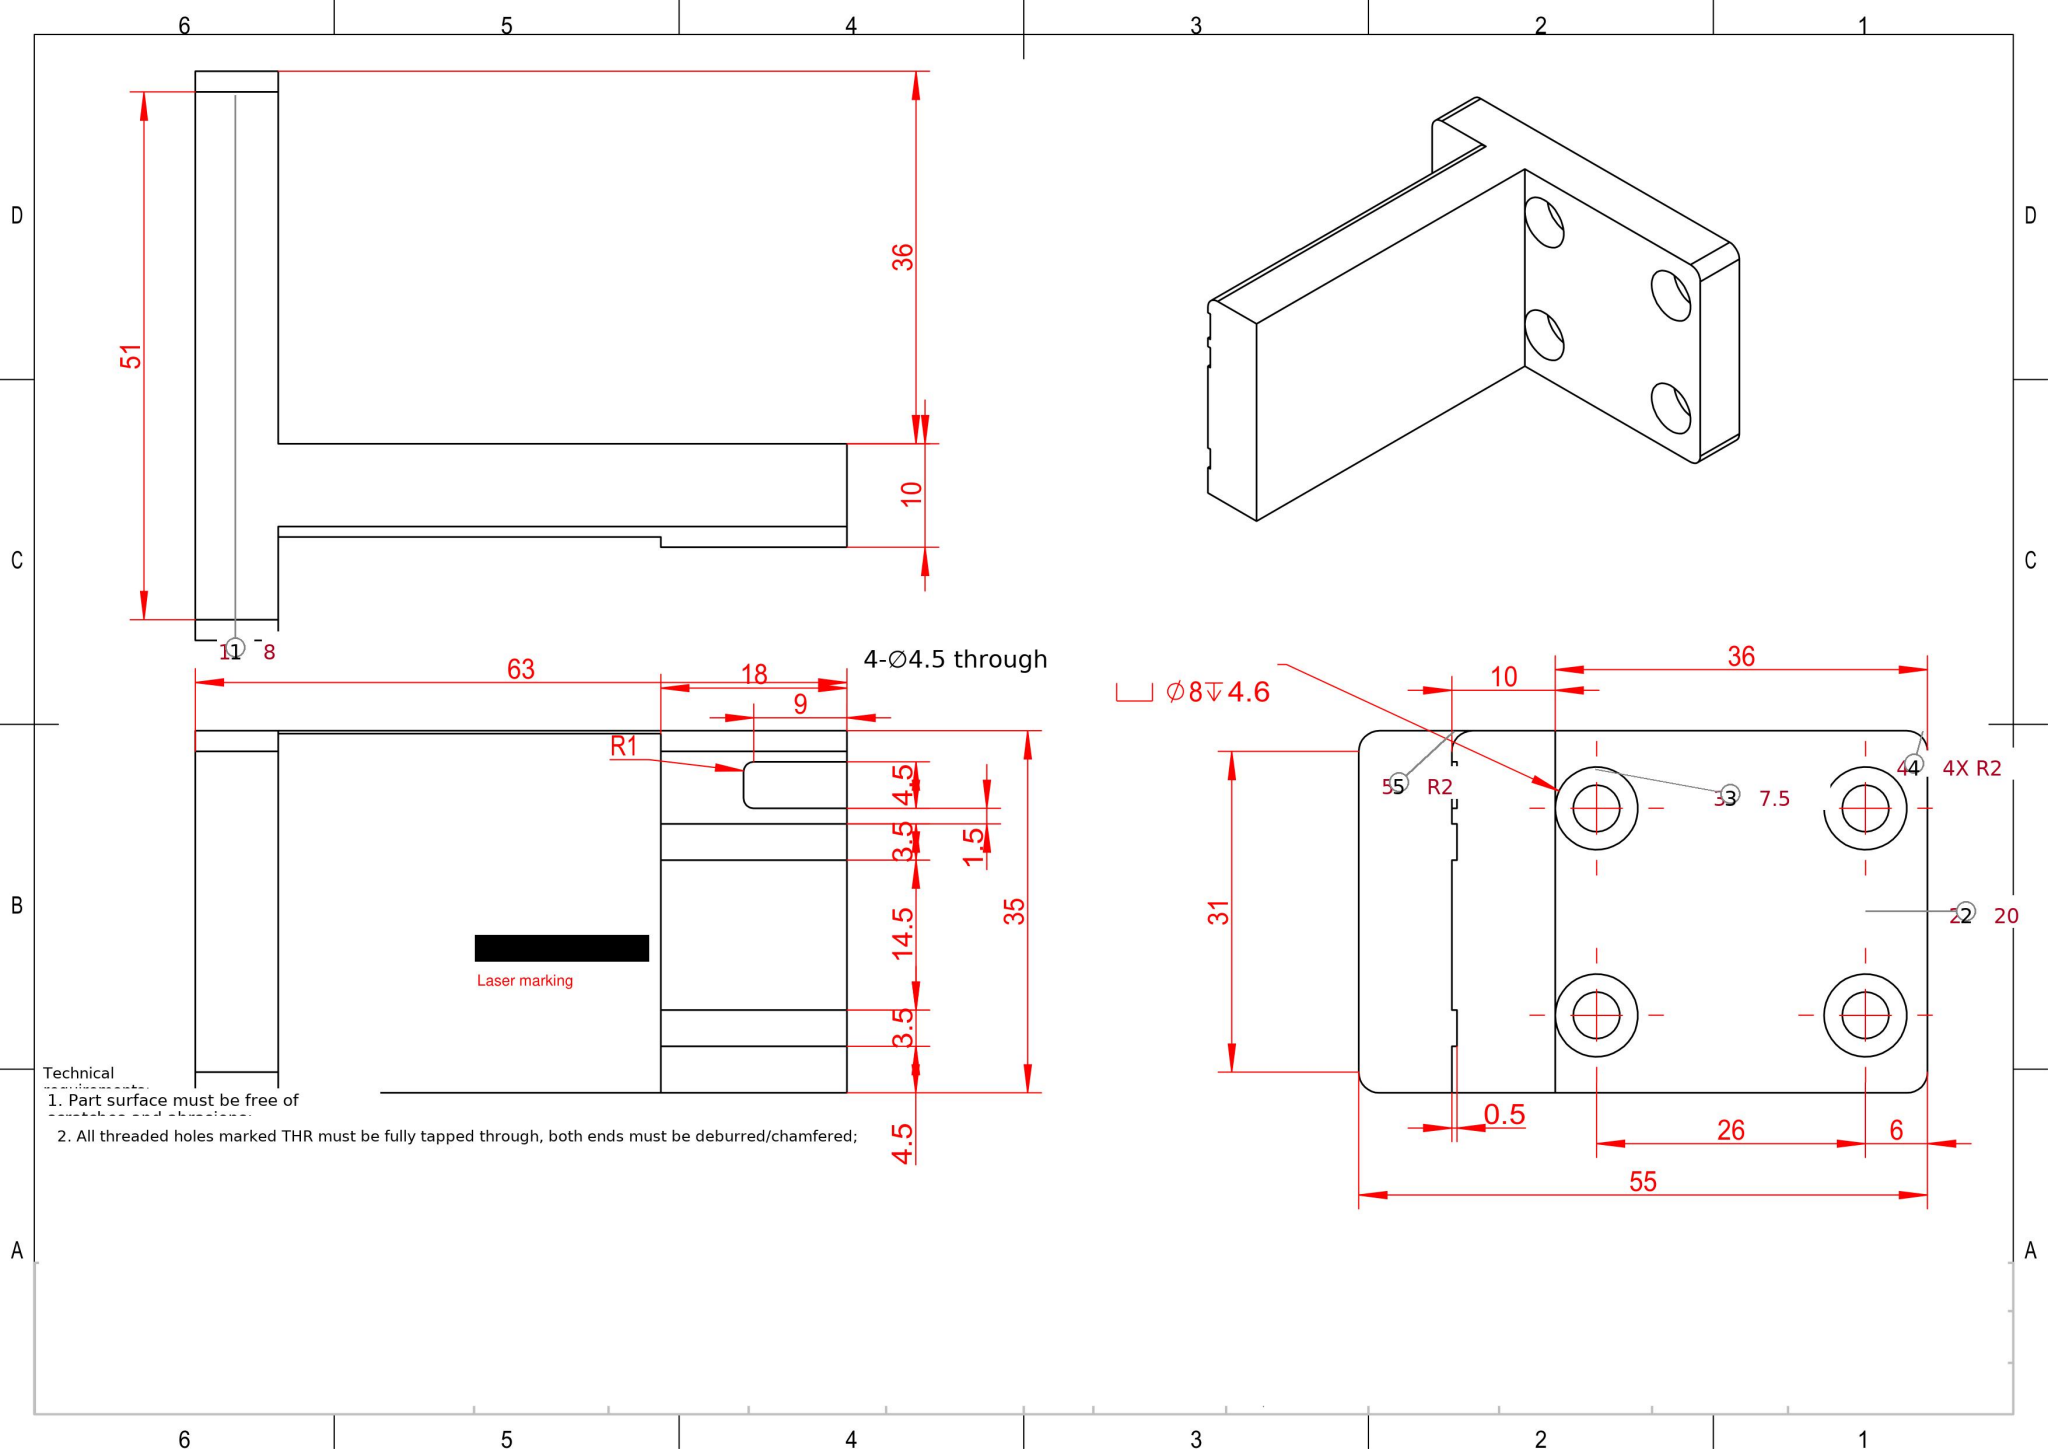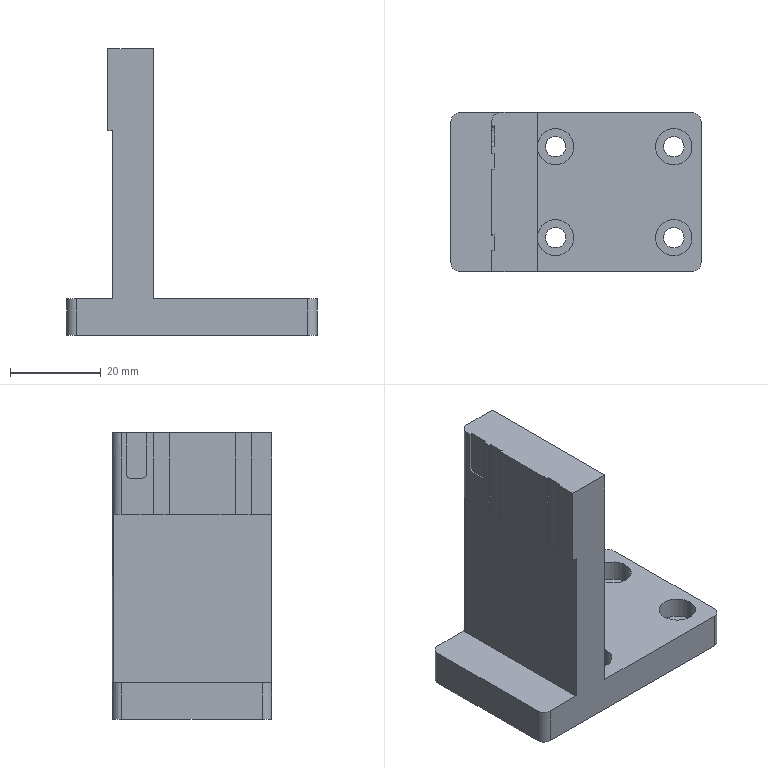Part | SolidWorks | mm | 1 solid | 51 faces | box 55 x 35 x 63 mm | volume 32082 mm3 | plane 28 | cylinder 23 | commonest cylinder face diameters 8 x8 4.5 x8 4 x5 2 x2